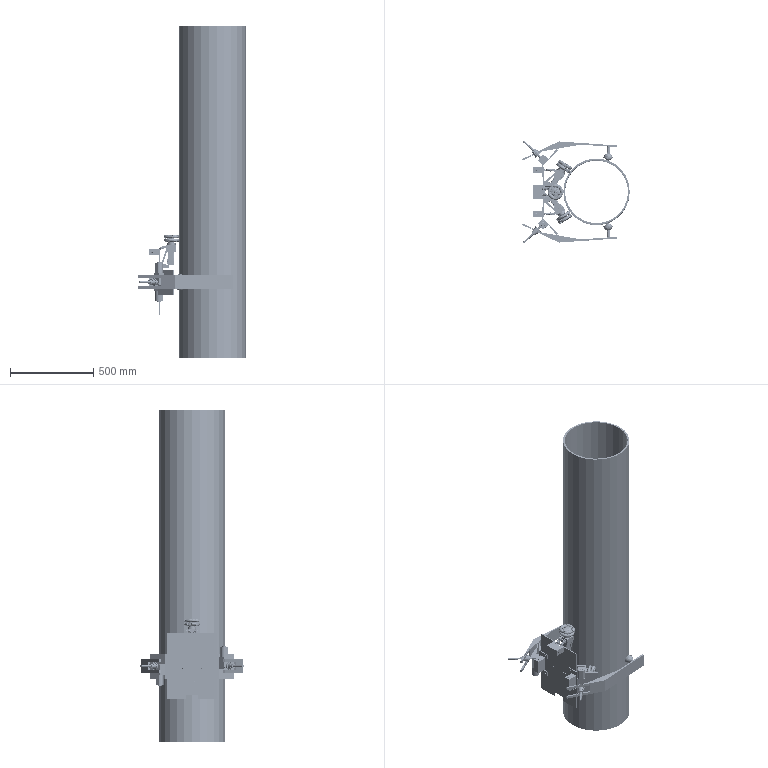Assembly | SolidWorks | mm | 79 component files | 89 solids | 6258 faces | box 647.51 x 623.31 x 2000 mm | volume 28803945 mm3 | plane 3134 | cylinder 2281 | cone 501 | torus 240 | sphere 90 | spline 12 | commonest cylinder face diameters 5 x200 3.236 x120 0.971 x120 9.223 x120 4 x96 6.472 x72 2.5 x68 10 x62
Bill of materials:
Chassis | 1 |  | Thin flat plate, roughly rectangular, with a rectangular notch cut into the middle of each of its four edges. It has four groups of four small through-holes, each group in a square pattern, and the groups sit in a diamond layout around the plate centre.
BallJoint | 2 |  | Solid sphere shown as a faceted surface mesh.
BallJointFixed | 2 |  | Flat annular ring (washer- or flange-like) with a large central bore and four equally spaced small through-holes near the outer edge. A narrower raised annular step stands out from one face.
BallJointSeat | 2 |  | Hemispherical dome joined to a thin circular flange at its open rim. A straight cylindrical stem sticks out from the dome apex along the axis. The flange has four equally spaced holes, and there are small notch or groove marks on the dome surface near the flange.
ClampingPlate | 2 |  | Flat bar bent at an obtuse angle. One end splits into a two-tine fork, and each tine has an elongated slot. There is a small hole near the bend, and the straight opposite end has a larger round through-hole.
ConnectingPinAxis | 2 |  | Long cylindrical rod with a rectangular flat plate attached along one side, tangent to the rod. The plate is shorter than the rod and has two round holes near its edge furthest from the rod.
LeadScrew | 2 |  | Straight solid cylindrical rod with a short reduced-diameter stepped end at one end. The other end is a plain flat face.
NutSeat | 2 |  | Flanged cylindrical body with a central through-bore that is counterbored or recessed at both ends. The circular flange has six larger bolt holes on a circle plus one smaller hole. A flat is cut along the side of the barrel, and it carries angled pockets or holes and small holes.
Sleeve | 2 |  | Short thin-walled cylindrical sleeve with a slender cylindrical pin passing straight through it, at right angles to the sleeve axis. The pin sticks out on both sides.
SupportPlate | 2 |  | Plate bent at an obtuse angle into two flat segments. One segment ends in a C-shaped cutout that leaves two rectangular tabs, each with two round holes. The other segment has two small holes near its edge.
WormGearMotor | 2 |  | Body with a square-section block at the bottom, a coaxial cylindrical section above it, and a small round boss on top. One side face of the block has a counterbored or bossed round hole between two small holes, and an adjacent face has two small holes near the bottom.
Pipe | 1 |  | Straight thin-walled round tube with open ends and constant diameter.
Bracket | 3 |  | Open rectangular box-like frame. The top and bottom walls have stepped notches, and the walls carry small holes, slots and a partial circular cutout.
ConnectingRod | 8 |  | Flat straight link bar with fully rounded ends and one through hole at each end.
ConnectingRodSeat | 3 |  | C-shaped bracket. A vertical back plate joins two tapered horizontal arms, and small cylindrical pins stick out from the arms.
CoverPlate | 2 |  | Flat rectangular plate with four corner through holes. A rectangular block sticks out from one face, giving a T-shaped side profile.
DamperBase | 3 |  | Straight square-section bar with four lugs on one side, arranged as two closely spaced pairs. Each lug has a rounded end and a through hole.
DamperBase2 | 3 |  | Block with two fork-like pairs of rounded-end lugs, each lug holed, on an angled body. The back face has two through holes.
DamperLowerEnd | 6 |  | Stepped turned shaft. A small pin end leads into a long cylindrical shank, a collar flange and a larger cylinder, which ends in a flat tab with a through-hole eye.
DamperUpperEnd | 6 |  | Short flanged cylindrical cup with a thin rod running along its axis. On the other side a tapered neck ends in a flat eye tab with a hole.
Motor | 3 |  | Assembly that looks like a motor with a geared output head. It has a long rectangular body, a square mounting flange with four corner holes, a round stepped housing with a screw circle, and an output shaft.
MotorBracket | 3 |  | Rectangular block with a large circular through bore. One face has four corner holes, short cylindrical pins stick out from top and bottom, and small holes sit on a side face.
Omni-directionalWheel | 3 |  | Wheel with a central hub and many barrel-shaped rollers around the rim. The rollers sit at an angle to the wheel axis, as on a mecanum-type wheel.
PressureSensor | 3 |  | Stepped solid cylinder: a large main body, a narrow circumferential groove, a flange of the same diameter, then two smaller concentric steps on one end face.
Spring | 4 |  | Open-pitch helical coil made of round-section wire. The coil diameter stays the same along its length, it has roughly 16-17 turns, and the overall cylindrical envelope is long compared to its diameter.
ConnectingRod2 | 2 |  | Straight, flat bar link of constant width and thickness. Both ends are fully rounded, and each end has one round through-hole.
ConnectingRod3 | 2 |  | Straight, flat bar link of constant width and thickness. Both ends are fully rounded, and each end has one round through-hole.
CoverPlate | 1 |  | Thin flat rectangular plate with four small through-holes near the corners, two rectangular notches cut into one long edge, and a single rectangular block or rib sticking out from the underside near the middle, giving a T-shaped side profile.
Spring | 2 |  | Cylindrical helical coil of round-section wire with roughly 14 to 16 closely spaced turns. The coil diameter looks constant, and the centre is open along the axis.
Mates:
1. coincident | Pipe-1 plane at (0, 0, 0) dir (0, 0, 1) | assembly plane at (0, 0, 0) dir (0, 0, 1)
2. coincident | Pipe-1 plane at (0, 0, 0) dir (0, 1, 0) | assembly plane at (0, 0, 0) dir (0, 1, 0)
3. coincident | Pipe-1 plane at (0, 0, 0) dir (1, 0, 0) | assembly plane at (0, 0, 0) dir (1, 0, 0)
4. coincident | Chassis-1 plane at (-320, 0, -542.97) dir (0, 1, 0) | assembly plane at (0, 0, 0) dir (0, 1, 0)
5. parallel | Chassis-1 face at (-320, 0, -542.97) dir (-1, 0, 0) | assembly plane at (0, 0, 0) dir (1, 0, 0)
6. coincident | WheelAssembly-1/Bracket-1 face at (-380, -113, -585.47) dir (-1, 0, 0) | WheelAssembly-2/Bracket-1 face at (-380, 113, -500.47) dir (-1, 0, 0)
7. coincident | Chassis-1 face at (-320, 0, -542.97) dir (-1, 0, 0) | WheelAssembly-2/Bracket-1 face at (-320, 113, -500.47) dir (1, 0, 0)
8. width | WheelAssembly-2/Bracket-1 face at (-350, 130.5, -500.47) dir (0, 0, 1) | WheelAssembly-2/Bracket-1 face at (-350, 130.5, -585.47) dir (0, 0, -1) | Chassis-1 face at (-315, 150, -742.97) dir (0, 0, -1) | Chassis-1 face at (-315, 150, -342.97) dir (0, 0, 1)
9. coincident | WheelAssembly-1/Bracket-1 face at (-350, -130.5, -500.47) dir (0, 0, 1) | WheelAssembly-2/Bracket-1 face at (-350, 130.5, -500.47) dir (0, 0, 1)
10. coincident | Chassis-1 face at (-315, -150, -342.97) dir (0, -1, 0) | WheelAssembly-1/CoverPlate-1 face at (-350, -150, -542.97) dir (0, -1, 0)
11. coincident | Chassis-1 face at (-315, 150, -342.97) dir (0, 1, 0) | WheelAssembly-2/CoverPlate-1 face at (-350, 150, -542.97) dir (0, 1, 0)
12. distance | assembly plane at (0, 0, 0) dir (1, 0, 0) | Chassis-1 face at (-320, 0, -542.97) dir (-1, 0, 0)
13. coincident | Chassis-1 face at (-320, 0, -542.97) dir (-1, 0, 0) | WheelAssembly2-1/Bracket-1 face at (-320, -42.5, -379.97) dir (1, 0, 0)
14. coincident | Chassis-1 face at (-315, 150, -342.97) dir (0, 0, 1) | WheelAssembly2-1/CoverPlate-1 face at (-350, 0, -342.97) dir (0, 0, 1)
15. width | WheelAssembly2-1/Bracket-1 face at (-350, 42.5, -362.47) dir (0, 1, 0) | WheelAssembly2-1/Bracket-1 face at (-350, -42.5, -362.47) dir (0, -1, 0) | Chassis-1 face at (-315, -150, -342.97) dir (0, -1, 0) | Chassis-1 face at (-315, 150, -342.97) dir (0, 1, 0)
16. coincident | ClampingMechanism-1/SupportPlate-1 face at (-326, -162.385, -467.97) dir (-1, 0, 0) | ClampingMechanism-2/SupportPlate-1 face at (-326, 162.385, -617.97) dir (-1, 0, 0)
17. coincident | ClampingMechanism-1/SupportPlate-1 face at (-235, -250, -467.97) dir (0, 0, 1) | ClampingMechanism-2/SupportPlate-1 face at (-235, 250, -467.97) dir (0, 0, 1)
18. coincident | Chassis-1 face at (-320, 0, -542.97) dir (-1, 0, 0) | ClampingMechanism-1/SupportPlate-1 face at (-320, -160, -467.97) dir (1, 0, 0)
19. width | ClampingMechanism-2/SupportPlate-1 face at (-235, 250, -617.97) dir (0, 0, -1) | ClampingMechanism-2/SupportPlate-1 face at (-235, 250, -467.97) dir (0, 0, 1) | Chassis-1 face at (-315, 150, -342.97) dir (0, 0, 1) | Chassis-1 face at (-315, 150, -742.97) dir (0, 0, -1)
20. coincident | WheelAssembly-1/CoverPlate-1 face at (-350, -150, -542.97) dir (0, -1, 0) | ClampingMechanism-1/SupportPlate-1 face at (-316, -150, -592.97) dir (0, 1, 0)
21. coincident | WheelAssembly-2/CoverPlate-1 face at (-350, 150, -542.97) dir (0, 1, 0) | ClampingMechanism-2/SupportPlate-1 face at (-316, 150, -492.97) dir (0, -1, 0)
22. angle | WheelAssembly-1/ConnectingRod-1 face at (-308.36, -64.703, -512.97) dir (-0.6719, -0.7406, 0) | Chassis-1 face at (-320, 0, -542.97) dir (-1, 0, 0)
23. angle | WheelAssembly-2/ConnectingRod-1 face at (-308.359, 64.704, -572.97) dir (-0.6717, 0.7408, 0) | Chassis-1 face at (-320, 0, -542.97) dir (-1, 0, 0)
24. angle | WheelAssembly2-1/ConnectingRod2-1 face at (-309.713, -33, -430.299) dir (-0.9425, 0, 0.3341) | Chassis-1 face at (-320, 0, -542.97) dir (-1, 0, 0)
25. tangent | Pipe-1 face at (0, 0, 1000) dir (0, 0, -1) r 200 | ClampingMechanism-1/BallJoint-1 face at (69.427, -208.758, -542.97) dir (1, 0, 0) r 20
26. tangent | Pipe-1 face at (0, 0, 1000) dir (0, 0, -1) r 200 | ClampingMechanism-2/BallJoint-1 face at (69.427, 208.758, -542.97) dir (1, 0, 0) r 20
27. coincident | SupportPlate-1 plane at (0, 0, 0) dir (0, 0, 1) | ClampingMechanism plane at (0, 0, 0) dir (0, 0, 1)
28. coincident | SupportPlate-1 plane at (0, 0, 0) dir (0, 1, 0) | ClampingMechanism plane at (0, 0, 0) dir (0, 1, 0)
29. coincident | SupportPlate-1 plane at (0, 0, 0) dir (1, 0, 0) | ClampingMechanism plane at (0, 0, 0) dir (1, 0, 0)
30. width | ClampingPlate-1 face at (-16.96, -358.774, 40) dir (0, 0, 1) | ClampingPlate-1 face at (-16.96, -358.774, -40) dir (0, 0, -1) | SupportPlate-1 face at (0, 0, -75) dir (0, 0, -1) | SupportPlate-1 face at (0, 0, 75) dir (0, 0, 1)
31. coincident | SupportPlate-1 face at (-4.12, 4.362, 75) dir (-0.6866, 0.727, 0) | WormGearMotor-1 face at (68.582, 73.024, 20.16) dir (0.6866, -0.727, 0)
32. concentric | WormGearMotor-1 edge at (39.743, 103.559, 0) dir (-0.6866, 0.727, 0) r 6 | LeadScrew-1 face at (-57.293, 206.304, 0) dir (0.6866, -0.727, 0) r 6
33. coincident | WormGearMotor-1 face at (45.7, 97.252, 39.435) dir (-0.6866, 0.727, 0) | LeadScrew-1 face at (45.7, 97.252, 0) dir (0.6866, -0.727, 0)
34. concentric | LeadScrew-1 face at (-57.293, 206.304, 0) dir (0.6866, -0.727, 0) r 6 | NutSeat-1 face at (-3.091, 148.913, 0) dir (-0.6866, 0.727, 0) r 14.25
35. distance | LeadScrew-1 face at (-57.293, 206.304, 0) dir (0.6866, -0.727, 0) r 6 | ClampingPlate-1 face at (-16.96, -358.774, 40) dir (0, 0, 1)
36. distance | LeadScrew-1 face at (-57.293, 206.304, 0) dir (0.6866, -0.727, 0) r 6 | SupportPlate-1 edge at (-4.12, 4.362, 75) dir (0, 0, -1)
37. parallel | SupportPlate-1 face at (-4.12, 4.362, 75) dir (-0.727, -0.6866, 0) | WormGearMotor-1 face at (23.668, 85.626, 56.16) dir (-0.727, -0.6866, 0)
38. concentric | NutSeat-1 face at (-3.091, 148.913, 0) dir (-0.6866, 0.727, 0) r 14.25 | Sleeve-1 face at (8.667, 136.463, 0) dir (0.6866, -0.727, 0) r 14.25
39. coincident | NutSeat-1 edge at (35.322, 134.128, -4.657) dir (-0.6866, 0.727, 0) r 2.062 | Sleeve-1 face at (22.399, 121.923, 0) dir (0.6866, -0.727, 0)
40. parallel | ClampingPlate-1 face at (-16.96, -358.774, 40) dir (0, 0, 1) | Sleeve-1 face at (15.533, 129.193, 40) dir (0, 0, 1)
41. tangent | ClampingPlate-1 face at (13.745, 119.536, -40) dir (-0.9046, 0.4263, 0) | Sleeve-1 face at (15.533, 129.193, -40) dir (0, 0, 1) r 2.5
42. concentric | ClampingPlate-1 face at (-24.355, -10.622, 30) dir (0, 0, 1) r 3 | ConnectingPinAxis-1 face at (-24.355, -10.622, 40) dir (0, 0, -1) r 3
43. coincident | ClampingPlate-1 face at (-16.96, -358.774, 40) dir (0, 0, 1) | ConnectingPinAxis-1 face at (-24.355, -10.622, 40) dir (0, 0, 1)
44. coincident | SupportPlate-1 face at (-4.12, 4.362, 75) dir (-0.6866, 0.727, 0) | ConnectingPinAxis-1 face at (-22.295, -12.804, 20) dir (0.6866, -0.727, 0)
45. distance | ConnectingPinAxis-1 face at (9.936, 25.89, 20) dir (0.727, 0.6866, 0) | SupportPlate-1 face at (-4.12, 4.362, 75) dir (-0.727, -0.6866, 0)
46. concentric | ClampingPlate-1 face at (-20.891, -308.929, 0) dir (-0.9969, -0.07862, 0) r 10 | BallJointSeat-1 face at (68.83, -301.853, 0) dir (0.9969, 0.07862, 0) r 10
47. coincident | ClampingPlate-1 face at (-26.929, -359.561, 40) dir (-0.9969, -0.07862, 0) | BallJointSeat-1 face at (-30.86, -309.715, 0) dir (-0.9969, -0.07862, 0)
48. concentric | BallJointSeat-1 face at (43.907, -303.819, 0) dir (1, 0, 0) r 20 | BallJoint-1 face at (43.907, -303.819, 0) dir (1, 0, 0) r 20
49. concentric | BallJointSeat-1 face at (38.923, -304.212, 0) dir (0.9969, 0.07862, 0) r 27.5 | BallJointFixed-1 face at (48.892, -303.426, 0) dir (-0.9969, -0.07862, 0) r 27.5
50. coincident | BallJointSeat-1 face at (43.907, -303.819, 0) dir (0.9969, 0.07862, 0) | BallJointFixed-1 face at (43.907, -303.819, 0) dir (-0.9969, -0.07862, 0)
51. concentric | BallJointSeat-1 face at (41.942, -278.896, 0) dir (0.9969, 0.07862, 0) r 1.25 | BallJointFixed-1 face at (41.942, -278.896, 0) dir (-0.9969, -0.07862, 0) r 1.25
52. coincident | Bracket-1 plane at (0, 0, 0) dir (0, 0, 1) | WheelAssembly plane at (0, 0, 0) dir (0, 0, 1)
53. coincident | Bracket-1 plane at (0, 0, 0) dir (0, 1, 0) | WheelAssembly plane at (0, 0, 0) dir (0, 1, 0)
54. coincident | Bracket-1 plane at (0, 0, 0) dir (1, 0, 0) | WheelAssembly plane at (0, 0, 0) dir (1, 0, 0)
55. coincident | Bracket-1 face at (17.5, 30, 42.5) dir (1, 0, 0) | CoverPlate-1 face at (17.5, 0, 0) dir (-1, 0, 0)
56. concentric | Bracket-1 face at (17.5, -26, -38.5) dir (1, 0, 0) r 1.25 | CoverPlate-1 face at (17.5, -26, -38.5) dir (1, 0, 0) r 2
57. coincident | Bracket-1 face at (-17.5, -30, 42.5) dir (0, -1, 0) | CoverPlate-1 face at (19.5, -30, 42.5) dir (0, -1, 0)
58. concentric | DamperUpperEnd-1 face at (8.396, -51.946, 17.5) dir (-0.2105, 0.9776, 0) r 1 | DamperLowerEnd-1 face at (4.582, -34.237, 17.5) dir (0.2105, -0.9776, 0) r 4
59. coincident | DamperUpperEnd-1 face at (-1.5, -6, 19) dir (0, 0, 1) | DamperLowerEnd-1 face at (14.372, -79.694, 19) dir (0, 0, 1)
60. concentric | Spring-1 face at (1.764, -21.153, 17.5) dir (-0.2105, 0.9776, 0) r 1.115 | DamperLowerEnd-1 face at (4.582, -34.237, 17.5) dir (0.2105, -0.9776, 0) r 4
61. coincident | Spring-1 face at (1.658, -20.664, 17.5) dir (-0.2105, 0.9776, 0) | DamperUpperEnd-1 face at (1.658, -20.664, 17.5) dir (0.2105, -0.9776, 0)
62. coincident | DamperUpperEnd-2 face at (-1.5, -6, -16) dir (0, 0, 1) | DamperLowerEnd-2 face at (14.372, -79.694, -16) dir (0, 0, 1)
63. concentric | DamperUpperEnd-2 face at (8.396, -51.946, -17.5) dir (-0.2105, 0.9776, 0) r 1 | DamperLowerEnd-2 face at (4.582, -34.237, -17.5) dir (0.2105, -0.9776, 0) r 4
64. coincident | DamperUpperEnd-2 face at (1.658, -20.664, -17.5) dir (0.2105, -0.9776, 0) | Spring-2 face at (1.658, -20.664, -17.5) dir (-0.2105, 0.9776, 0)
65. concentric | DamperLowerEnd-2 face at (4.582, -34.237, -17.5) dir (0.2105, -0.9776, 0) r 4 | Spring-2 face at (1.764, -21.153, -17.5) dir (-0.2105, 0.9776, 0) r 1.115
66. concentric | DamperUpperEnd-1 face at (-1.5, -6, 16) dir (0, 0, 1) r 2 | DamperUpperEnd-2 face at (-1.5, -6, -19) dir (0, 0, 1) r 2
67. concentric | DamperLowerEnd-1 face at (14.372, -79.694, 19) dir (0, 0, -1) r 2.5 | DamperLowerEnd-2 face at (14.372, -79.694, -16) dir (0, 0, -1) r 2.5
68. coincident | Bracket-1 face at (2.5, 10, -57.5) dir (-1, 0, 0) | DamperBase-1 face at (2.5, 10, 42.5) dir (1, 0, 0)
69. coincident | Bracket-1 face at (0, 0, 42.5) dir (0, 0, 1) | DamperBase-1 face at (-1.5, 6, 42.5) dir (0, 0, 1)
70. concentric | DamperUpperEnd-1 face at (-1.5, -6, 16) dir (0, 0, 1) r 2 | DamperBase-1 edge at (-1.5, -6, 15) dir (0, 0, -1) r 2
71. width | DamperUpperEnd-1 face at (-1.5, -6, 19) dir (0, 0, 1) | DamperUpperEnd-1 face at (-1.5, -6, 16) dir (0, 0, -1) | DamperBase-1 face at (-6.5, 2, 10) dir (0, 0, -1) | DamperBase-1 face at (-1.5, -6, 25) dir (0, 0, 1)
72. width | DamperUpperEnd-2 face at (-1.5, -6, -16) dir (0, 0, 1) | DamperUpperEnd-2 face at (-1.5, -6, -19) dir (0, 0, -1) | DamperBase-1 face at (-1.5, -6, -25) dir (0, 0, -1) | DamperBase-1 face at (-6.5, 2, -10) dir (0, 0, 1)
73. concentric | DamperLowerEnd-1 face at (14.372, -79.694, 19) dir (0, 0, -1) r 2.5 | DamperBase2-1 face at (14.372, -79.694, 25) dir (0, 0, -1) r 2
74. coincident | DamperBase-1 face at (-1.5, -6, 25) dir (0, 0, 1) | DamperBase2-1 face at (14.372, -79.694, 25) dir (0, 0, 1)
75. concentric | Omni-directionalWheel-1 face at (77.312, -169.041, 0) dir (-0.8511, 0.525, 0) r 7.5 | Motor-1 face at (-1.82, -120.229, 0) dir (-0.8511, 0.525, 0) r 7.5
76. coincident | Omni-directionalWheel-1 face at (16.564, -131.569, 0) dir (-0.8511, 0.525, 0) | Motor-1 face at (25.746, -116.683, 0) dir (0.8511, -0.525, 0)
77. concentric | Motor-1 face at (-1.82, -120.229, 0) dir (-0.8511, 0.525, 0) r 25.2 | MotorBracket-1 face at (2.436, -122.854, 0) dir (-0.8511, 0.525, 0) r 25.5
78. coincident | Motor-1 face at (9.874, -101.272, 22.274) dir (0.8511, -0.525, 0) | MotorBracket-1 face at (-1.82, -120.229, 0) dir (-0.8511, 0.525, 0)
79. parallel | Motor-1 face at (7.249, -94.099, 22.274) dir (0.525, 0.8511, 0) | MotorBracket-1 face at (18.186, -97.321, -30) dir (0.525, 0.8511, 0)
80. coincident | DamperBase2-1 face at (7.547, -90.759, 0) dir (-0.525, -0.8511, 0) | MotorBracket-1 face at (18.186, -97.321, -30) dir (0.525, 0.8511, 0)
81. width | MotorBracket-1 face at (18.186, -97.321, 30) dir (0, 0, 1) | MotorBracket-1 face at (18.186, -97.321, -30) dir (0, 0, -1) | DamperBase2-1 face at (13.079, -94.171, -25) dir (0, 0, -1) | DamperBase2-1 face at (14.372, -79.694, 25) dir (0, 0, 1)
82. width | DamperBase2-1 face at (3.59, -84.793, 25) dir (-0.8511, 0.525, 0) | DamperBase2-1 face at (19.904, -83.107, 25) dir (0.8511, -0.525, 0) | MotorBracket-1 face at (2.436, -122.854, 0) dir (0.8511, -0.525, 0) | MotorBracket-1 face at (-18.842, -109.729, 0) dir (-0.8511, 0.525, 0)
83. concentric | ConnectingRod-1 face at (-69.5, -45, -30) dir (0, 0, -1) r 2.5 | ConnectingRod-2 face at (-69.5, -45, 33) dir (0, 0, -1) r 2.5
84. concentric | ConnectingRod-1 face at (2.297, -99.27, -30) dir (0, 0, -1) r 2.5 | ConnectingRod-2 face at (2.297, -99.27, 33) dir (0, 0, -1) r 2.5
85. concentric | ConnectingRod-3 face at (-90.5, -79.044, 33) dir (0, 0, -1) r 2.5 | ConnectingRod-4 face at (-90.5, -79.044, -30) dir (0, 0, -1) r 2.5
86. concentric | ConnectingRod-3 face at (-18.703, -133.314, 33) dir (0, 0, -1) r 2.5 | ConnectingRod-4 face at (-18.703, -133.314, -30) dir (0, 0, -1) r 2.5
87. concentric | MotorBracket-1 face at (2.297, -99.27, 35) dir (0, 0, -1) r 2.5 | ConnectingRod-2 face at (2.297, -99.27, 33) dir (0, 0, -1) r 2.5
88. coincident | MotorBracket-1 face at (18.186, -97.321, -30) dir (0, 0, -1) | ConnectingRod-1 face at (-69.5, -45, -30) dir (0, 0, 1)
89. concentric | MotorBracket-1 face at (-18.703, -133.314, 35) dir (0, 0, -1) r 2.5 | ConnectingRod-4 face at (-18.703, -133.314, -30) dir (0, 0, -1) r 2.5
90. coincident | ConnectingRod-2 face at (-69.5, -45, 33) dir (0, 0, 1) | ConnectingRod-3 face at (-90.5, -79.044, 33) dir (0, 0, 1)
91. coincident | MotorBracket-1 face at (18.186, -97.321, 30) dir (0, 0, 1) | ConnectingRod-2 face at (-69.5, -45, 30) dir (0, 0, -1)
92. coincident | ConnectingRod-1 face at (-69.5, -45, -30) dir (0, 0, 1) | ConnectingRod-4 face at (-90.5, -79.044, -30) dir (0, 0, 1)
93. concentric | ConnectingRod-2 face at (-69.5, -45, 33) dir (0, 0, -1) r 2.5 | ConnectingRodSeat-1 face at (-69.5, -45, 35) dir (0, 0, -1) r 2.5
94. concentric | ConnectingRod-3 face at (-90.5, -79.044, 33) dir (0, 0, -1) r 2.5 | ConnectingRodSeat-1 face at (-90.5, -79.044, 35) dir (0, 0, -1) r 2.5
95. coincident | ConnectingRod-2 edge at (-69.5, -45, 30) dir (0, 0, 1) r 5 | ConnectingRodSeat-1 face at (-97.5, -90, 30) dir (0, 0, 1)
96. distance | ConnectingRodSeat-1 face at (-97.5, -35, 35) dir (0, 1, 0) | Bracket-1 face at (-17.5, -30, 42.5) dir (0, -1, 0)
97. distance | ConnectingRodSeat-1 edge at (-62.5, -35, 0) dir (1, 0, 0) | Bracket-1 face at (17.5, 30, 42.5) dir (1, 0, 0)
98. distance | Bracket-1 face at (-17.5, 30, 42.5) dir (0, 1, 0) | PressureSensor-1 face at (1, 26, 0) dir (0, 1, 0)
99. concentric | Bracket-1 face at (1, 26, 0) dir (0, -1, 0) r 10 | PressureSensor-1 face at (1, 13, 0) dir (0, 1, 0) r 10
100. concentric | Bracket-1 face at (-6.5, 30, 0) dir (0, -1, 0) r 1.5 | PressureSensor-1 face at (-6.5, 26, 0) dir (0, 1, 0) r 0.8
101. coincident | Bracket-1 face at (-5.5, 2, -57.5) dir (0, 1, 0) | DamperBase-1 face at (-5.5, 2, 42.5) dir (0, -1, 0)
102. coincident | Bracket-1 plane at (0, 0, 0) dir (0, 0, 1) | WheelAssembly2 plane at (0, 0, 0) dir (0, 0, 1)
103. coincident | Bracket-1 plane at (0, 0, 0) dir (0, 1, 0) | WheelAssembly2 plane at (0, 0, 0) dir (0, 1, 0)
104. coincident | Bracket-1 plane at (0, 0, 0) dir (1, 0, 0) | WheelAssembly2 plane at (0, 0, 0) dir (1, 0, 0)
105. coincident | Bracket-1 face at (17.5, 30, 42.5) dir (1, 0, 0) | CoverPlate-1 face at (17.5, 0, 0) dir (-1, 0, 0)
106. concentric | Bracket-1 face at (17.5, -26, -38.5) dir (1, 0, 0) r 1.25 | CoverPlate-1 face at (17.5, -26, -38.5) dir (1, 0, 0) r 2
107. coincident | Bracket-1 face at (-17.5, -30, 42.5) dir (0, -1, 0) | CoverPlate-1 face at (19.5, -30, 42.5) dir (0, -1, 0)
108. concentric | DamperUpperEnd-1 face at (10.49, -51.445, 17.5) dir (-0.2551, 0.9669, 0) r 1 | DamperLowerEnd-1 face at (7.47, -40, 17.5) dir (0.2551, -0.9669, 0) r 4
109. coincident | DamperUpperEnd-1 face at (-1.5, -6, 19) dir (0, 0, 1) | DamperLowerEnd-1 face at (19.332, -84.961, 19) dir (0, 0, 1)
110. concentric | Spring-1 face at (2.411, -20.824, 17.5) dir (-0.2551, 0.9669, 0) r 1.115 | DamperLowerEnd-1 face at (7.47, -40, 17.5) dir (0.2551, -0.9669, 0) r 4
111. coincident | Spring-1 face at (2.326, -20.504, 17.5) dir (-0.2551, 0.9669, 0) | DamperUpperEnd-1 face at (2.326, -20.504, 17.5) dir (0.2551, -0.9669, 0)
112. coincident | DamperUpperEnd-2 face at (-1.5, -6, -16) dir (0, 0, 1) | DamperLowerEnd-2 face at (19.332, -84.961, -16) dir (0, 0, 1)
113. concentric | DamperUpperEnd-2 face at (10.49, -51.445, -17.5) dir (-0.2551, 0.9669, 0) r 1 | DamperLowerEnd-2 face at (7.47, -40, -17.5) dir (0.2551, -0.9669, 0) r 4
114. coincident | DamperUpperEnd-2 face at (2.326, -20.504, -17.5) dir (0.2551, -0.9669, 0) | Spring-2 face at (2.326, -20.504, -17.5) dir (-0.2551, 0.9669, 0)
115. concentric | DamperLowerEnd-2 face at (7.47, -40, -17.5) dir (0.2551, -0.9669, 0) r 4 | Spring-2 face at (2.411, -20.824, -17.5) dir (-0.2551, 0.9669, 0) r 1.115
116. concentric | DamperUpperEnd-1 face at (-1.5, -6, 16) dir (0, 0, 1) r 2 | DamperUpperEnd-2 face at (-1.5, -6, -19) dir (0, 0, 1) r 2
117. concentric | DamperLowerEnd-1 face at (19.332, -84.961, 19) dir (0, 0, -1) r 2.5 | DamperLowerEnd-2 face at (19.332, -84.961, -16) dir (0, 0, -1) r 2.5
118. coincident | Bracket-1 face at (2.5, 10, -57.5) dir (-1, 0, 0) | DamperBase-1 face at (2.5, 10, 42.5) dir (1, 0, 0)
119. coincident | Bracket-1 face at (0, 0, 42.5) dir (0, 0, 1) | DamperBase-1 face at (-1.5, 6, 42.5) dir (0, 0, 1)
120. concentric | DamperUpperEnd-1 face at (-1.5, -6, 16) dir (0, 0, 1) r 2 | DamperBase-1 edge at (-1.5, -6, 15) dir (0, 0, -1) r 2
121. width | DamperUpperEnd-1 face at (-1.5, -6, 19) dir (0, 0, 1) | DamperUpperEnd-1 face at (-1.5, -6, 16) dir (0, 0, -1) | DamperBase-1 face at (-6.5, 2, 10) dir (0, 0, -1) | DamperBase-1 face at (-1.5, -6, 25) dir (0, 0, 1)
122. width | DamperUpperEnd-2 face at (-1.5, -6, -16) dir (0, 0, 1) | DamperUpperEnd-2 face at (-1.5, -6, -19) dir (0, 0, -1) | DamperBase-1 face at (-1.5, -6, -25) dir (0, 0, -1) | DamperBase-1 face at (-6.5, 2, -10) dir (0, 0, 1)
123. concentric | DamperLowerEnd-1 face at (19.332, -84.961, 19) dir (0, 0, -1) r 2.5 | DamperBase2-1 face at (19.332, -84.961, 25) dir (0, 0, -1) r 2
124. coincident | DamperBase-1 face at (-1.5, -6, 25) dir (0, 0, 1) | DamperBase2-1 face at (19.332, -84.961, 25) dir (0, 0, 1)
125. concentric | Omni-directionalWheel-1 face at (120.077, -127.326, 0) dir (-1, -0.006314, 0) r 7.5 | Motor-1 face at (27.103, -127.913, 0) dir (-1, -0.006314, 0) r 7.5
126. coincident | Omni-directionalWheel-1 face at (48.703, -127.776, 0) dir (-1, -0.006314, 0) | Motor-1 face at (48.593, -110.287, 0) dir (1, 0.006314, 0)
127. concentric | Motor-1 face at (27.103, -127.913, 0) dir (-1, -0.006314, 0) r 25.2 | MotorBracket-1 face at (32.103, -127.881, 0) dir (-1, -0.006314, 0) r 25.5
128. coincident | Motor-1 face at (26.963, -105.639, 22.274) dir (1, 0.006314, 0) | MotorBracket-1 face at (27.103, -127.913, 0) dir (-1, -0.006314, 0)
129. parallel | Motor-1 face at (20.933, -100.951, 22.274) dir (-0.006314, 1, 0) | MotorBracket-1 face at (31.914, -97.882, -30) dir (-0.006314, 1, 0)
130. coincident | DamperBase2-1 face at (19.414, -97.961, 0) dir (0.006314, -1, 0) | MotorBracket-1 face at (31.914, -97.882, -30) dir (-0.006314, 1, 0)
131. width | MotorBracket-1 face at (31.914, -97.882, 30) dir (0, 0, 1) | MotorBracket-1 face at (31.914, -97.882, -30) dir (0, 0, -1) | DamperBase2-1 face at (25.914, -97.92, -25) dir (0, 0, -1) | DamperBase2-1 face at (19.332, -84.961, 25) dir (0, 0, 1)
132. width | DamperBase2-1 face at (12.895, -95.002, 25) dir (-1, -0.006314, 0) | DamperBase2-1 face at (25.832, -84.92, 25) dir (1, 0.006314, 0) | MotorBracket-1 face at (32.103, -127.881, 0) dir (1, 0.006314, 0) | MotorBracket-1 face at (7.104, -128.039, 0) dir (-1, -0.006314, 0)
133. distance | ConnectingRodSeat-1 face at (-97.5, -35, 35) dir (0, 1, 0) | Bracket-1 face at (-17.5, -30, 42.5) dir (0, -1, 0)
134. distance | ConnectingRodSeat-1 edge at (-62.5, -35, 0) dir (1, 0, 0) | Bracket-1 face at (17.5, 30, 42.5) dir (1, 0, 0)
135. distance | Bracket-1 face at (-17.5, 30, 42.5) dir (0, 1, 0) | PressureSensor-1 face at (1, 26, 0) dir (0, 1, 0)
136. concentric | Bracket-1 face at (1, 26, 0) dir (0, -1, 0) r 10 | PressureSensor-1 face at (1, 13, 0) dir (0, 1, 0) r 10
137. concentric | Bracket-1 face at (-6.5, 30, 0) dir (0, -1, 0) r 1.5 | PressureSensor-1 face at (-6.5, 26, 0) dir (0, 1, 0) r 0.8
138. concentric | ConnectingRod2-1 face at (-69.5, -45, 33) dir (0, 0, -1) r 2.5 | ConnectingRod2-2 face at (-69.5, -45, -30) dir (0, 0, -1) r 2.5
139. concentric | ConnectingRod2-1 face at (19.477, -107.961, 33) dir (0, 0, -1) r 2.5 | ConnectingRod2-2 face at (19.477, -107.961, -30) dir (0, 0, -1) r 2.5
140. concentric | MotorBracket-1 face at (19.477, -107.961, 35) dir (0, 0, -1) r 2.5 | ConnectingRod2-2 face at (19.477, -107.961, -30) dir (0, 0, -1) r 2.5
141. coincident | MotorBracket-1 face at (31.914, -97.882, 30) dir (0, 0, 1) | ConnectingRod2-1 face at (-69.5, -45, 30) dir (0, 0, -1)
142. coincident | MotorBracket-1 face at (31.914, -97.882, -30) dir (0, 0, -1) | ConnectingRod2-2 face at (-69.5, -45, -30) dir (0, 0, 1)
143. concentric | ConnectingRodSeat-1 face at (-69.5, -45, 35) dir (0, 0, -1) r 2.5 | ConnectingRod2-1 face at (-69.5, -45, 33) dir (0, 0, -1) r 2.5
144. concentric | ConnectingRod3-1 face at (-90.5, -79.044, 33) dir (0, 0, -1) r 2.5 | ConnectingRod3-2 face at (-90.5, -79.044, -30) dir (0, 0, -1) r 2.5
145. concentric | ConnectingRod3-1 face at (19.73, -147.96, 33) dir (0, 0, -1) r 2.5 | ConnectingRod3-2 face at (19.73, -147.96, -30) dir (0, 0, -1) r 2.5
146. concentric | MotorBracket-1 face at (19.73, -147.96, 35) dir (0, 0, -1) r 2.5 | ConnectingRod3-2 face at (19.73, -147.96, -30) dir (0, 0, -1) r 2.5
147. coincident | MotorBracket-1 face at (31.914, -97.882, -30) dir (0, 0, -1) | ConnectingRod3-2 face at (-90.5, -79.044, -30) dir (0, 0, 1)
148. coincident | ConnectingRod2-1 face at (-69.5, -45, 33) dir (0, 0, 1) | ConnectingRod3-1 face at (-90.5, -79.044, 33) dir (0, 0, 1)
149. concentric | ConnectingRodSeat-1 face at (-90.5, -79.044, 35) dir (0, 0, -1) r 2.5 | ConnectingRod3-1 face at (-90.5, -79.044, 33) dir (0, 0, -1) r 2.5
150. coincident | ConnectingRodSeat-1 face at (-97.5, -90, 30) dir (0, 0, 1) | ConnectingRod2-1 face at (-69.5, -45, 30) dir (0, 0, -1)
151. coincident | Bracket-1 face at (-5.5, 2, -57.5) dir (0, 1, 0) | DamperBase-1 face at (-5.5, 2, 42.5) dir (0, -1, 0)